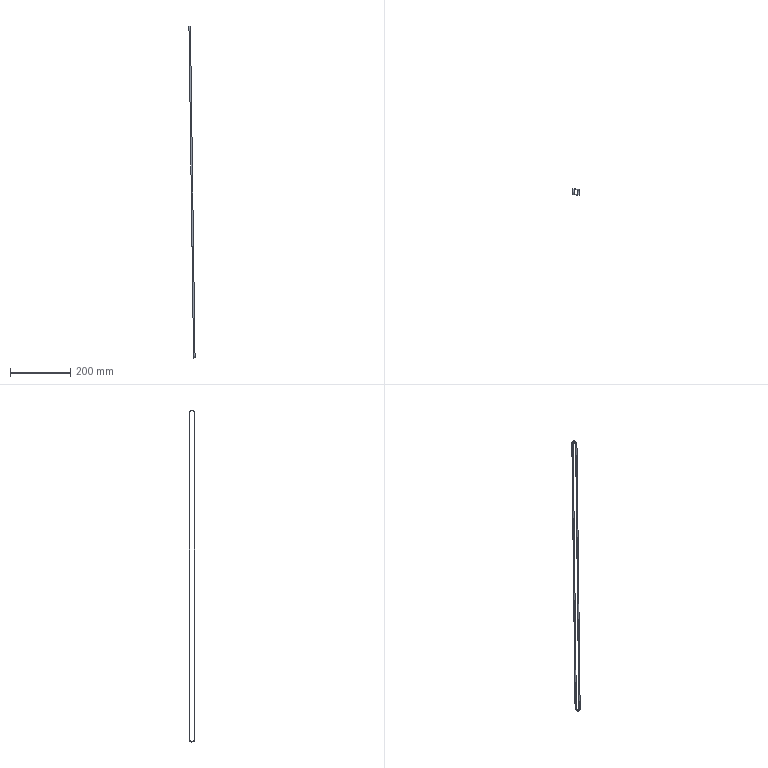Component | SolidWorks | DA-0220-Part16-3 | 1 solid | 12 faces | box 20.34 x 19.01 x 1098.96 mm | volume 13849 mm3 | cylinder 6 | plane 6 | commonest cylinder face diameters 16.5 x3 19 x3
build123d program:
from build123d import *

# Parameters (mm, degrees)
THICKEN_THIN1_DEPTH = 5


with BuildPart() as part:
    # Sketch1 → Thicken-Thin1 (new body)
    with BuildSketch(Plane.XY):
        with BuildLine():
            Line((540, -9.5), (-540, -9.5))
            ThreePointArc((-540, -9.5), (-549.5, 0), (-540, 9.5))
            Line((-540, 9.5), (540, 9.5))
            ThreePointArc((540, 9.5), (549.5, 0), (540, -9.5))
        make_face()
        with BuildLine():
            Line((540, -8.25), (-540, -8.25))
            ThreePointArc((-540, -8.25), (-548.25, 0), (-540, 8.25))
            Line((-540, 8.25), (540, 8.25))
            ThreePointArc((540, 8.25), (548.25, 0), (540, -8.25))
        make_face(mode=Mode.SUBTRACT)
    extrude(amount=-THICKEN_THIN1_DEPTH)


solid = part.part

# Placed as in the assembly
solid = solid.moved(Location((1002.058, -33.647, 17.485), (-1.659, 89.2, -178.341)))
STEP:
#1=COLOUR_RGB('',0.7922,0.8196,0.9333);
#2=FILL_AREA_STYLE_COLOUR('',#1);
#3=FILL_AREA_STYLE('',(#2));
#4=SURFACE_STYLE_FILL_AREA(#3);
#5=SURFACE_SIDE_STYLE('',(#4));
#6=SURFACE_STYLE_USAGE(.BOTH.,#5);
#7=PRESENTATION_STYLE_ASSIGNMENT((#6));
#8=CARTESIAN_POINT('',(38.953,-1.325,22.268));
#9=VERTEX_POINT('',#8);
#10=CARTESIAN_POINT('',(38.958,-1.65,21.943));
#11=VERTEX_POINT('',#10);
#12=CARTESIAN_POINT('',(38.958,-1.325,21.943));
#13=DIRECTION('',(0.9999,0.000404,0.01395));
#14=DIRECTION('',(-0.01395,-0.00000282,0.9999));
#15=AXIS2_PLACEMENT_3D('',#12,#13,#14);
#16=CIRCLE('',#15,0.3248);
#17=EDGE_CURVE('',#9,#11,#16,.T.);
#18=ORIENTED_EDGE('',*,*,#17,.F.);
#19=CARTESIAN_POINT('',(39.15,-1.325,22.271));
#20=VERTEX_POINT('',#19);
#21=CARTESIAN_POINT('',(38.953,-1.325,22.268));
#22=DIRECTION('',(0.9999,0.000404,0.01395));
#23=VECTOR('',#22,39.37);
#24=LINE('',#21,#23);
#25=EDGE_CURVE('',#9,#20,#24,.T.);
#26=ORIENTED_EDGE('',*,*,#25,.T.);
#27=CARTESIAN_POINT('',(39.155,-1.65,21.946));
#28=VERTEX_POINT('',#27);
#29=CARTESIAN_POINT('',(39.154,-1.325,21.946));
#30=DIRECTION('',(0.9999,0.000404,0.01395));
#31=DIRECTION('',(-0.01395,-0.00000282,0.9999));
#32=AXIS2_PLACEMENT_3D('',#29,#30,#31);
#33=CIRCLE('',#32,0.3248);
#34=EDGE_CURVE('',#20,#28,#33,.T.);
#35=ORIENTED_EDGE('',*,*,#34,.T.);
#36=CARTESIAN_POINT('',(38.958,-1.65,21.943));
#37=DIRECTION('',(0.9999,0.000404,0.01395));
#38=VECTOR('',#37,39.37);
#39=LINE('',#36,#38);
#40=EDGE_CURVE('',#11,#28,#39,.T.);
#41=ORIENTED_EDGE('',*,*,#40,.F.);
#42=EDGE_LOOP('',(#18,#26,#35,#41));
#43=FACE_OUTER_BOUND('',#42,.T.);
#44=CARTESIAN_POINT('',(38.958,-1.325,21.943));
#45=DIRECTION('',(0.9999,0.000404,0.01395));
#46=DIRECTION('',(-0.01395,-0.00000282,0.9999));
#47=AXIS2_PLACEMENT_3D('',#44,#45,#46);
#48=CYLINDRICAL_SURFACE('',#47,0.3248);
#49=ADVANCED_FACE('',(#43),#48,.F.);
#50=CARTESIAN_POINT('',(38.957,-0.9508,21.943));
#51=VERTEX_POINT('',#50);
#52=CARTESIAN_POINT('',(38.952,-1.325,22.317));
#53=VERTEX_POINT('',#52);
#54=CARTESIAN_POINT('',(38.958,-1.325,21.943));
#55=DIRECTION('',(0.9999,0.000404,0.01395));
#56=DIRECTION('',(-0.01395,-0.00000282,0.9999));
#57=AXIS2_PLACEMENT_3D('',#54,#55,#56);
#58=CIRCLE('',#57,0.374);
#59=EDGE_CURVE('',#51,#53,#58,.T.);
#60=ORIENTED_EDGE('',*,*,#59,.T.);
#61=CARTESIAN_POINT('',(39.149,-1.325,22.32));
#62=VERTEX_POINT('',#61);
#63=CARTESIAN_POINT('',(38.952,-1.325,22.317));
#64=DIRECTION('',(0.9999,0.000404,0.01395));
#65=VECTOR('',#64,39.37);
#66=LINE('',#63,#65);
#67=EDGE_CURVE('',#53,#62,#66,.T.);
#68=ORIENTED_EDGE('',*,*,#67,.T.);
#69=CARTESIAN_POINT('',(39.154,-0.9507,21.946));
#70=VERTEX_POINT('',#69);
#71=CARTESIAN_POINT('',(39.154,-1.325,21.946));
#72=DIRECTION('',(0.9999,0.000404,0.01395));
#73=DIRECTION('',(-0.01395,-0.00000282,0.9999));
#74=AXIS2_PLACEMENT_3D('',#71,#72,#73);
#75=CIRCLE('',#74,0.374);
#76=EDGE_CURVE('',#70,#62,#75,.T.);
#77=ORIENTED_EDGE('',*,*,#76,.F.);
#78=CARTESIAN_POINT('',(38.957,-0.9508,21.943));
#79=DIRECTION('',(0.9999,0.000404,0.01395));
#80=VECTOR('',#79,39.37);
#81=LINE('',#78,#80);
#82=EDGE_CURVE('',#51,#70,#81,.T.);
#83=ORIENTED_EDGE('',*,*,#82,.F.);
#84=EDGE_LOOP('',(#60,#68,#77,#83));
#85=FACE_OUTER_BOUND('',#84,.T.);
#86=CARTESIAN_POINT('',(38.958,-1.325,21.943));
#87=DIRECTION('',(0.9999,0.000404,0.01395));
#88=DIRECTION('',(-0.01395,-0.00000282,0.9999));
#89=AXIS2_PLACEMENT_3D('',#86,#87,#88);
#90=CYLINDRICAL_SURFACE('',#89,0.374);
#91=ADVANCED_FACE('',(#85),#90,.T.);
#92=CARTESIAN_POINT('',(39.748,-1.699,-20.569));
#93=VERTEX_POINT('',#92);
#94=CARTESIAN_POINT('',(39.748,-0.9506,-20.569));
#95=VERTEX_POINT('',#94);
#96=CARTESIAN_POINT('',(39.748,-1.325,-20.569));
#97=DIRECTION('',(0.9999,0.000404,0.01395));
#98=DIRECTION('',(-0.01395,-0.00000282,0.9999));
#99=AXIS2_PLACEMENT_3D('',#96,#97,#98);
#100=CIRCLE('',#99,0.374);
#101=EDGE_CURVE('',#93,#95,#100,.T.);
#102=ORIENTED_EDGE('',*,*,#101,.F.);
#103=CARTESIAN_POINT('',(39.551,-1.699,-20.572));
#104=VERTEX_POINT('',#103);
#105=CARTESIAN_POINT('',(39.551,-1.699,-20.572));
#106=DIRECTION('',(0.9999,0.000404,0.01395));
#107=VECTOR('',#106,39.37);
#108=LINE('',#105,#107);
#109=EDGE_CURVE('',#104,#93,#108,.T.);
#110=ORIENTED_EDGE('',*,*,#109,.F.);
#111=CARTESIAN_POINT('',(39.551,-0.9507,-20.572));
#112=VERTEX_POINT('',#111);
#113=CARTESIAN_POINT('',(39.551,-1.325,-20.572));
#114=DIRECTION('',(0.9999,0.000404,0.01395));
#115=DIRECTION('',(-0.01395,-0.00000282,0.9999));
#116=AXIS2_PLACEMENT_3D('',#113,#114,#115);
#117=CIRCLE('',#116,0.374);
#118=EDGE_CURVE('',#104,#112,#117,.T.);
#119=ORIENTED_EDGE('',*,*,#118,.T.);
#120=CARTESIAN_POINT('',(39.551,-0.9507,-20.572));
#121=DIRECTION('',(0.9999,0.000404,0.01395));
#122=VECTOR('',#121,39.37);
#123=LINE('',#120,#122);
#124=EDGE_CURVE('',#112,#95,#123,.T.);
#125=ORIENTED_EDGE('',*,*,#124,.T.);
#126=EDGE_LOOP('',(#102,#110,#119,#125));
#127=FACE_OUTER_BOUND('',#126,.T.);
#128=CARTESIAN_POINT('',(39.551,-1.325,-20.572));
#129=DIRECTION('',(0.9999,0.000404,0.01395));
#130=DIRECTION('',(-0.01395,-0.00000282,0.9999));
#131=AXIS2_PLACEMENT_3D('',#128,#129,#130);
#132=CYLINDRICAL_SURFACE('',#131,0.374);
#133=ADVANCED_FACE('',(#127),#132,.T.);
#134=CARTESIAN_POINT('',(39.155,-1.699,21.946));
#135=VERTEX_POINT('',#134);
#136=CARTESIAN_POINT('',(39.748,-1.699,-20.569));
#137=DIRECTION('',(0.01395,0.00000282,-0.9999));
#138=VECTOR('',#137,39.37);
#139=LINE('',#136,#138);
#140=EDGE_CURVE('',#135,#93,#139,.T.);
#141=ORIENTED_EDGE('',*,*,#140,.F.);
#142=CARTESIAN_POINT('',(38.958,-1.699,21.943));
#143=VERTEX_POINT('',#142);
#144=CARTESIAN_POINT('',(38.958,-1.699,21.943));
#145=DIRECTION('',(0.9999,0.000404,0.01395));
#146=VECTOR('',#145,39.37);
#147=LINE('',#144,#146);
#148=EDGE_CURVE('',#143,#135,#147,.T.);
#149=ORIENTED_EDGE('',*,*,#148,.F.);
#150=CARTESIAN_POINT('',(39.551,-1.699,-20.572));
#151=DIRECTION('',(0.01395,0.00000282,-0.9999));
#152=VECTOR('',#151,39.37);
#153=LINE('',#150,#152);
#154=EDGE_CURVE('',#143,#104,#153,.T.);
#155=ORIENTED_EDGE('',*,*,#154,.T.);
#156=ORIENTED_EDGE('',*,*,#109,.T.);
#157=EDGE_LOOP('',(#141,#149,#155,#156));
#158=FACE_OUTER_BOUND('',#157,.T.);
#159=CARTESIAN_POINT('',(39.551,-1.699,-20.572));
#160=DIRECTION('',(0.000404,-1.,0.00000282));
#161=DIRECTION('',(0.01395,0.00000282,-0.9999));
#162=AXIS2_PLACEMENT_3D('',#159,#160,#161);
#163=PLANE('',#162);
#164=ADVANCED_FACE('',(#158),#163,.T.);
#165=ORIENTED_EDGE('',*,*,#67,.F.);
#166=CARTESIAN_POINT('',(38.958,-1.325,21.943));
#167=DIRECTION('',(0.9999,0.000404,0.01395));
#168=DIRECTION('',(-0.01395,-0.00000282,0.9999));
#169=AXIS2_PLACEMENT_3D('',#166,#167,#168);
#170=CIRCLE('',#169,0.374);
#171=EDGE_CURVE('',#53,#143,#170,.T.);
#172=ORIENTED_EDGE('',*,*,#171,.T.);
#173=ORIENTED_EDGE('',*,*,#148,.T.);
#174=CARTESIAN_POINT('',(39.154,-1.325,21.946));
#175=DIRECTION('',(0.9999,0.000404,0.01395));
#176=DIRECTION('',(-0.01395,-0.00000282,0.9999));
#177=AXIS2_PLACEMENT_3D('',#174,#175,#176);
#178=CIRCLE('',#177,0.374);
#179=EDGE_CURVE('',#62,#135,#178,.T.);
#180=ORIENTED_EDGE('',*,*,#179,.F.);
#181=EDGE_LOOP('',(#165,#172,#173,#180));
#182=FACE_OUTER_BOUND('',#181,.T.);
#183=CARTESIAN_POINT('',(38.958,-1.325,21.943));
#184=DIRECTION('',(0.9999,0.000404,0.01395));
#185=DIRECTION('',(-0.01395,-0.00000282,0.9999));
#186=AXIS2_PLACEMENT_3D('',#183,#184,#185);
#187=CYLINDRICAL_SURFACE('',#186,0.374);
#188=ADVANCED_FACE('',(#182),#187,.T.);
#189=CARTESIAN_POINT('',(39.748,-0.9506,-20.569));
#190=DIRECTION('',(-0.01395,-0.00000282,0.9999));
#191=VECTOR('',#190,39.37);
#192=LINE('',#189,#191);
#193=EDGE_CURVE('',#95,#70,#192,.T.);
#194=ORIENTED_EDGE('',*,*,#193,.F.);
#195=ORIENTED_EDGE('',*,*,#124,.F.);
#196=CARTESIAN_POINT('',(39.551,-0.9507,-20.572));
#197=DIRECTION('',(-0.01395,-0.00000282,0.9999));
#198=VECTOR('',#197,39.37);
#199=LINE('',#196,#198);
#200=EDGE_CURVE('',#112,#51,#199,.T.);
#201=ORIENTED_EDGE('',*,*,#200,.T.);
#202=ORIENTED_EDGE('',*,*,#82,.T.);
#203=EDGE_LOOP('',(#194,#195,#201,#202));
#204=FACE_OUTER_BOUND('',#203,.T.);
#205=CARTESIAN_POINT('',(39.551,-0.9507,-20.572));
#206=DIRECTION('',(-0.000404,1.,-0.00000282));
#207=DIRECTION('',(-0.01395,-0.00000282,0.9999));
#208=AXIS2_PLACEMENT_3D('',#205,#206,#207);
#209=PLANE('',#208);
#210=ADVANCED_FACE('',(#204),#209,.T.);
#211=CARTESIAN_POINT('',(39.551,-1.65,-20.572));
#212=VERTEX_POINT('',#211);
#213=CARTESIAN_POINT('',(39.551,-1.65,-20.572));
#214=DIRECTION('',(0.01395,0.00000282,-0.9999));
#215=VECTOR('',#214,39.37);
#216=LINE('',#213,#215);
#217=EDGE_CURVE('',#11,#212,#216,.T.);
#218=ORIENTED_EDGE('',*,*,#217,.T.);
#219=CARTESIAN_POINT('',(39.551,-0.9999,-20.572));
#220=VERTEX_POINT('',#219);
#221=CARTESIAN_POINT('',(39.551,-1.325,-20.572));
#222=DIRECTION('',(0.9999,0.000404,0.01395));
#223=DIRECTION('',(-0.01395,-0.00000282,0.9999));
#224=AXIS2_PLACEMENT_3D('',#221,#222,#223);
#225=CIRCLE('',#224,0.3248);
#226=EDGE_CURVE('',#212,#220,#225,.T.);
#227=ORIENTED_EDGE('',*,*,#226,.T.);
#228=CARTESIAN_POINT('',(38.957,-1.,21.943));
#229=VERTEX_POINT('',#228);
#230=CARTESIAN_POINT('',(39.551,-0.9999,-20.572));
#231=DIRECTION('',(-0.01395,-0.00000282,0.9999));
#232=VECTOR('',#231,39.37);
#233=LINE('',#230,#232);
#234=EDGE_CURVE('',#220,#229,#233,.T.);
#235=ORIENTED_EDGE('',*,*,#234,.T.);
#236=CARTESIAN_POINT('',(38.958,-1.325,21.943));
#237=DIRECTION('',(0.9999,0.000404,0.01395));
#238=DIRECTION('',(-0.01395,-0.00000282,0.9999));
#239=AXIS2_PLACEMENT_3D('',#236,#237,#238);
#240=CIRCLE('',#239,0.3248);
#241=EDGE_CURVE('',#229,#9,#240,.T.);
#242=ORIENTED_EDGE('',*,*,#241,.T.);
#243=ORIENTED_EDGE('',*,*,#17,.T.);
#244=EDGE_LOOP('',(#218,#227,#235,#242,#243));
#245=FACE_BOUND('',#244,.T.);
#246=ORIENTED_EDGE('',*,*,#118,.F.);
#247=ORIENTED_EDGE('',*,*,#154,.F.);
#248=ORIENTED_EDGE('',*,*,#171,.F.);
#249=ORIENTED_EDGE('',*,*,#59,.F.);
#250=ORIENTED_EDGE('',*,*,#200,.F.);
#251=EDGE_LOOP('',(#246,#247,#248,#249,#250));
#252=FACE_OUTER_BOUND('',#251,.T.);
#253=CARTESIAN_POINT('',(39.551,-1.325,-20.572));
#254=DIRECTION('',(0.9999,0.000404,0.01395));
#255=DIRECTION('',(-0.01395,-0.00000282,0.9999));
#256=AXIS2_PLACEMENT_3D('',#253,#254,#255);
#257=PLANE('',#256);
#258=ADVANCED_FACE('',(#245,#252),#257,.F.);
#259=CARTESIAN_POINT('',(39.748,-1.649,-20.569));
#260=VERTEX_POINT('',#259);
#261=CARTESIAN_POINT('',(39.748,-0.9998,-20.569));
#262=VERTEX_POINT('',#261);
#263=CARTESIAN_POINT('',(39.748,-1.325,-20.569));
#264=DIRECTION('',(0.9999,0.000404,0.01395));
#265=DIRECTION('',(-0.01395,-0.00000282,0.9999));
#266=AXIS2_PLACEMENT_3D('',#263,#264,#265);
#267=CIRCLE('',#266,0.3248);
#268=EDGE_CURVE('',#260,#262,#267,.T.);
#269=ORIENTED_EDGE('',*,*,#268,.F.);
#270=CARTESIAN_POINT('',(39.748,-1.649,-20.569));
#271=DIRECTION('',(0.01395,0.00000282,-0.9999));
#272=VECTOR('',#271,39.37);
#273=LINE('',#270,#272);
#274=EDGE_CURVE('',#28,#260,#273,.T.);
#275=ORIENTED_EDGE('',*,*,#274,.F.);
#276=ORIENTED_EDGE('',*,*,#34,.F.);
#277=CARTESIAN_POINT('',(39.154,-1.,21.946));
#278=VERTEX_POINT('',#277);
#279=CARTESIAN_POINT('',(39.154,-1.325,21.946));
#280=DIRECTION('',(0.9999,0.000404,0.01395));
#281=DIRECTION('',(-0.01395,-0.00000282,0.9999));
#282=AXIS2_PLACEMENT_3D('',#279,#280,#281);
#283=CIRCLE('',#282,0.3248);
#284=EDGE_CURVE('',#278,#20,#283,.T.);
#285=ORIENTED_EDGE('',*,*,#284,.F.);
#286=CARTESIAN_POINT('',(39.748,-0.9998,-20.569));
#287=DIRECTION('',(-0.01395,-0.00000282,0.9999));
#288=VECTOR('',#287,39.37);
#289=LINE('',#286,#288);
#290=EDGE_CURVE('',#262,#278,#289,.T.);
#291=ORIENTED_EDGE('',*,*,#290,.F.);
#292=EDGE_LOOP('',(#269,#275,#276,#285,#291));
#293=FACE_BOUND('',#292,.T.);
#294=ORIENTED_EDGE('',*,*,#101,.T.);
#295=ORIENTED_EDGE('',*,*,#193,.T.);
#296=ORIENTED_EDGE('',*,*,#76,.T.);
#297=ORIENTED_EDGE('',*,*,#179,.T.);
#298=ORIENTED_EDGE('',*,*,#140,.T.);
#299=EDGE_LOOP('',(#294,#295,#296,#297,#298));
#300=FACE_OUTER_BOUND('',#299,.T.);
#301=CARTESIAN_POINT('',(39.748,-1.325,-20.569));
#302=DIRECTION('',(0.9999,0.000404,0.01395));
#303=DIRECTION('',(-0.01395,-0.00000282,0.9999));
#304=AXIS2_PLACEMENT_3D('',#301,#302,#303);
#305=PLANE('',#304);
#306=ADVANCED_FACE('',(#293,#300),#305,.T.);
#307=ORIENTED_EDGE('',*,*,#268,.T.);
#308=CARTESIAN_POINT('',(39.551,-0.9999,-20.572));
#309=DIRECTION('',(0.9999,0.000404,0.01395));
#310=VECTOR('',#309,39.37);
#311=LINE('',#308,#310);
#312=EDGE_CURVE('',#220,#262,#311,.T.);
#313=ORIENTED_EDGE('',*,*,#312,.F.);
#314=ORIENTED_EDGE('',*,*,#226,.F.);
#315=CARTESIAN_POINT('',(39.551,-1.65,-20.572));
#316=DIRECTION('',(0.9999,0.000404,0.01395));
#317=VECTOR('',#316,39.37);
#318=LINE('',#315,#317);
#319=EDGE_CURVE('',#212,#260,#318,.T.);
#320=ORIENTED_EDGE('',*,*,#319,.T.);
#321=EDGE_LOOP('',(#307,#313,#314,#320));
#322=FACE_OUTER_BOUND('',#321,.T.);
#323=CARTESIAN_POINT('',(39.551,-1.325,-20.572));
#324=DIRECTION('',(0.9999,0.000404,0.01395));
#325=DIRECTION('',(-0.01395,-0.00000282,0.9999));
#326=AXIS2_PLACEMENT_3D('',#323,#324,#325);
#327=CYLINDRICAL_SURFACE('',#326,0.3248);
#328=ADVANCED_FACE('',(#322),#327,.F.);
#329=ORIENTED_EDGE('',*,*,#274,.T.);
#330=ORIENTED_EDGE('',*,*,#319,.F.);
#331=ORIENTED_EDGE('',*,*,#217,.F.);
#332=ORIENTED_EDGE('',*,*,#40,.T.);
#333=EDGE_LOOP('',(#329,#330,#331,#332));
#334=FACE_OUTER_BOUND('',#333,.T.);
#335=CARTESIAN_POINT('',(39.551,-1.65,-20.572));
#336=DIRECTION('',(0.000404,-1.,0.00000282));
#337=DIRECTION('',(0.01395,0.00000282,-0.9999));
#338=AXIS2_PLACEMENT_3D('',#335,#336,#337);
#339=PLANE('',#338);
#340=ADVANCED_FACE('',(#334),#339,.F.);
#341=ORIENTED_EDGE('',*,*,#25,.F.);
#342=ORIENTED_EDGE('',*,*,#241,.F.);
#343=CARTESIAN_POINT('',(38.957,-1.,21.943));
#344=DIRECTION('',(0.9999,0.000404,0.01395));
#345=VECTOR('',#344,39.37);
#346=LINE('',#343,#345);
#347=EDGE_CURVE('',#229,#278,#346,.T.);
#348=ORIENTED_EDGE('',*,*,#347,.T.);
#349=ORIENTED_EDGE('',*,*,#284,.T.);
#350=EDGE_LOOP('',(#341,#342,#348,#349));
#351=FACE_OUTER_BOUND('',#350,.T.);
#352=CARTESIAN_POINT('',(38.958,-1.325,21.943));
#353=DIRECTION('',(0.9999,0.000404,0.01395));
#354=DIRECTION('',(-0.01395,-0.00000282,0.9999));
#355=AXIS2_PLACEMENT_3D('',#352,#353,#354);
#356=CYLINDRICAL_SURFACE('',#355,0.3248);
#357=ADVANCED_FACE('',(#351),#356,.F.);
#358=ORIENTED_EDGE('',*,*,#290,.T.);
#359=ORIENTED_EDGE('',*,*,#347,.F.);
#360=ORIENTED_EDGE('',*,*,#234,.F.);
#361=ORIENTED_EDGE('',*,*,#312,.T.);
#362=EDGE_LOOP('',(#358,#359,#360,#361));
#363=FACE_OUTER_BOUND('',#362,.T.);
#364=CARTESIAN_POINT('',(39.551,-0.9999,-20.572));
#365=DIRECTION('',(-0.000404,1.,-0.00000282));
#366=DIRECTION('',(-0.01395,-0.00000282,0.9999));
#367=AXIS2_PLACEMENT_3D('',#364,#365,#366);
#368=PLANE('',#367);
#369=ADVANCED_FACE('',(#363),#368,.F.);
#370=CLOSED_SHELL('',(#49,#91,#133,#164,#188,#210,#258,#306,#328,#340,#357,#369));
#371=MANIFOLD_SOLID_BREP('',#370);
#372=STYLED_ITEM('',(#7),#371);
#373=(LENGTH_UNIT()NAMED_UNIT(*)SI_UNIT($,.METRE.));
#374=LENGTH_MEASURE_WITH_UNIT(LENGTH_MEASURE(0.0254),#373);
#375=DIMENSIONAL_EXPONENTS(1.,0.,0.,0.,0.,0.,0.);
#376=(CONVERSION_BASED_UNIT('',#374)LENGTH_UNIT()NAMED_UNIT(#375));
#377=UNCERTAINTY_MEASURE_WITH_UNIT(LENGTH_MEASURE(0.00001),#376,'','');
#378=(NAMED_UNIT(*)PLANE_ANGLE_UNIT()SI_UNIT($,.RADIAN.));
#379=(NAMED_UNIT(*)SI_UNIT($,.STERADIAN.)SOLID_ANGLE_UNIT());
#380=(GEOMETRIC_REPRESENTATION_CONTEXT(3)GLOBAL_UNCERTAINTY_ASSIGNED_CONTEXT((#377))GLOBAL_UNIT_ASSIGNED_CONTEXT((#376,#378,#379))REPRESENTATION_CONTEXT('',''));
#381=MECHANICAL_DESIGN_GEOMETRIC_PRESENTATION_REPRESENTATION('',(#372),#380);
#382=CARTESIAN_POINT('',(0.,0.,0.));
#383=DIRECTION('',(0.,0.,1.));
#384=DIRECTION('',(1.,0.,0.));
#385=AXIS2_PLACEMENT_3D('',#382,#383,#384);
#386=(LENGTH_UNIT()NAMED_UNIT(*)SI_UNIT($,.METRE.));
#387=LENGTH_MEASURE_WITH_UNIT(LENGTH_MEASURE(0.0254),#386);
#388=DIMENSIONAL_EXPONENTS(1.,0.,0.,0.,0.,0.,0.);
#389=(CONVERSION_BASED_UNIT('',#387)LENGTH_UNIT()NAMED_UNIT(#388));
#390=UNCERTAINTY_MEASURE_WITH_UNIT(LENGTH_MEASURE(0.00001),#389,'','');
#391=(NAMED_UNIT(*)PLANE_ANGLE_UNIT()SI_UNIT($,.RADIAN.));
#392=(NAMED_UNIT(*)SI_UNIT($,.STERADIAN.)SOLID_ANGLE_UNIT());
#393=(GEOMETRIC_REPRESENTATION_CONTEXT(3)GLOBAL_UNCERTAINTY_ASSIGNED_CONTEXT((#390))GLOBAL_UNIT_ASSIGNED_CONTEXT((#389,#391,#392))REPRESENTATION_CONTEXT('',''));
#394=ADVANCED_BREP_SHAPE_REPRESENTATION('',(#371,#385),#393);
#395=PRESENTATION_LAYER_ASSIGNMENT('','',(#372));